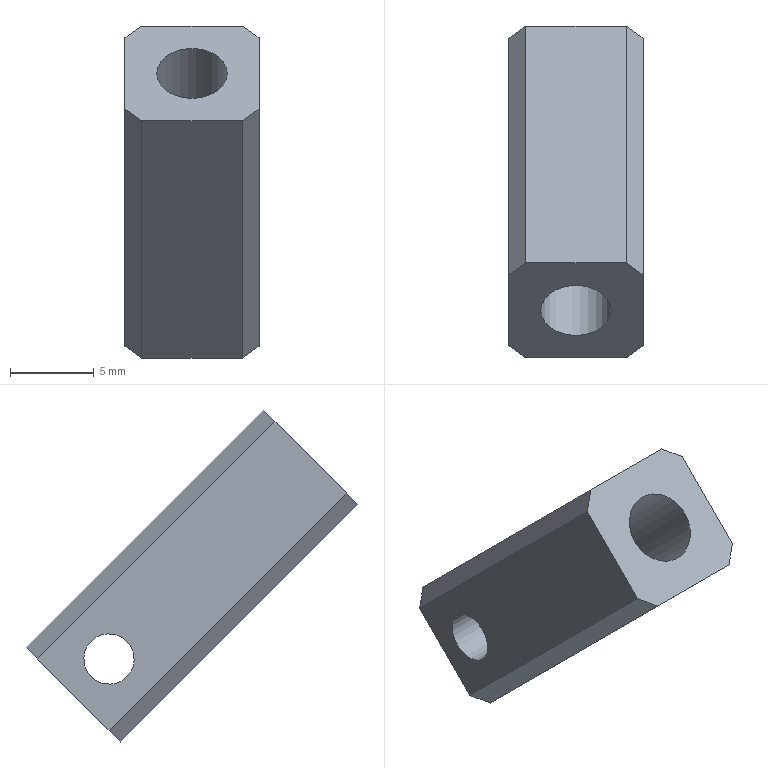Component | SolidWorks | ZL-10-08FloatingJoint-1 | 1 solid | 16 faces | box 8 x 19.8 x 19.8 mm | volume 1006 mm3 | plane 10 | cylinder 4 | cone 2 | commonest cylinder face diameters 3 x2 4.2 x2
build123d program:
from build123d import *

# Parameters (mm, degrees)
SKETCH1_W             = 8
SKETCH1_H             = 8
EXTRUDE1_DEPTH        = 20
M5_TAPPED_HOLE1_D     = 4.2
M5_TAPPED_HOLE1_DEPTH = 12.4
M5_TAPPED_HOLE1_TIP   = 1.262
SKETCH4_R             = 1.5
CUT_EXTRUDE1_DEPTH    = 22.909
CHAMFER1_SIZE         = 1


with BuildPart() as part:
    # Sketch1 → Extrude1 (new body)
    with BuildSketch(Plane.XY):
        Rectangle(SKETCH1_W, SKETCH1_H)
    extrude(amount=-EXTRUDE1_DEPTH)

    # M5 Tapped Hole1
    with Locations(Plane.XY):
        with Locations((0, 0)):
            Hole(M5_TAPPED_HOLE1_D / 2, depth=M5_TAPPED_HOLE1_DEPTH)
            with Locations((0, 0, -(M5_TAPPED_HOLE1_DEPTH + M5_TAPPED_HOLE1_TIP / 2))):  # 118° drill point
                Cone(0, M5_TAPPED_HOLE1_D / 2, M5_TAPPED_HOLE1_TIP, mode=Mode.SUBTRACT)

    # Sketch4 → Cut-Extrude1 (cut, through all)
    with BuildSketch(Plane(origin=(4, 0, 0), x_dir=(0, 0, -1), z_dir=(1, 0, 0))):
        with Locations(Location((17, 0, 0), (0, 0, 90))):
            Circle(SKETCH4_R)
    extrude(amount=-CUT_EXTRUDE1_DEPTH, mode=Mode.SUBTRACT)

    # Chamfer1
    chamfer1_edges = [part.edges().sort_by_distance(p)[0] for p in [
        (-4, 4, -10),
        (4, 4, -10),
        (4, -4, -10),
        (-4, -4, -10),
    ]]
    chamfer(chamfer1_edges, length=CHAMFER1_SIZE)


solid = part.part

# Placed as in the assembly
solid = solid.moved(Location((42.823, 52.548, -7.213), (45, 0, -180)))